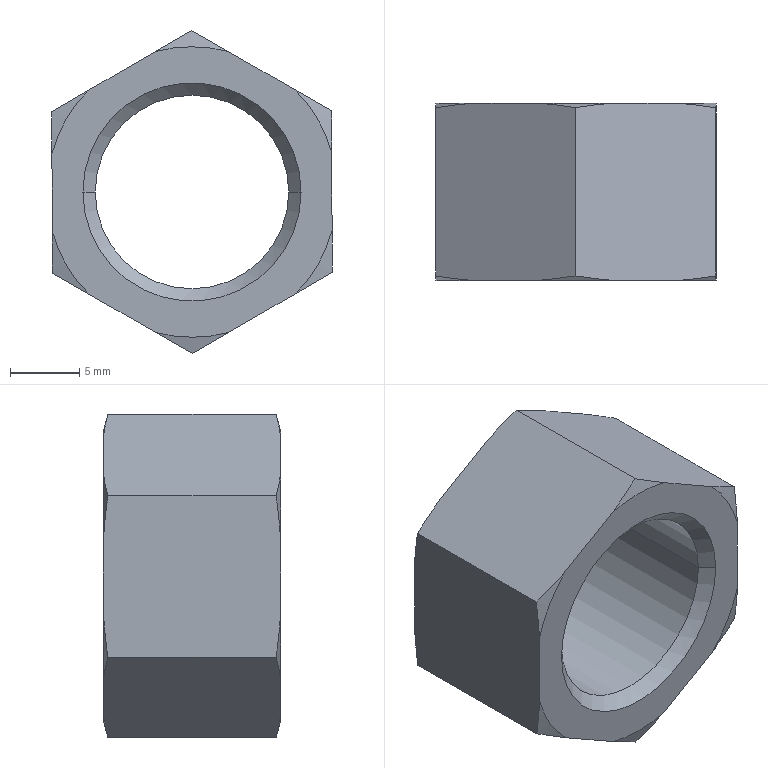Component | SolidWorks | 25Type1HexNut_GradeAAndB[GBT6170-2000][M14]-2 | 1 solid | 26 faces | box 20.28 x 12.8 x 23.36 mm | volume 2527 mm3 | cone 16 | plane 8 | cylinder 2 | commonest cylinder face diameters 14 x2 | material Steel
STEP:
#1=COLOUR_RGB('',0.7922,0.8196,0.9333);
#2=FILL_AREA_STYLE_COLOUR('',#1);
#3=FILL_AREA_STYLE('',(#2));
#4=SURFACE_STYLE_FILL_AREA(#3);
#5=SURFACE_SIDE_STYLE('',(#4));
#6=SURFACE_STYLE_USAGE(.BOTH.,#5);
#7=PRESENTATION_STYLE_ASSIGNMENT((#6));
#8=CARTESIAN_POINT('',(4.247,3.56,16.299));
#9=VERTEX_POINT('',#8);
#10=CARTESIAN_POINT('',(4.799,3.56,16.299));
#11=VERTEX_POINT('',#10);
#12=CARTESIAN_POINT('',(4.523,3.56,16.299));
#13=DIRECTION('',(-0.,1.,0.));
#14=DIRECTION('',(-1.,0.,0.));
#15=AXIS2_PLACEMENT_3D('',#12,#13,#14);
#16=CIRCLE('',#15,0.2756);
#17=EDGE_CURVE('',#9,#11,#16,.T.);
#18=ORIENTED_EDGE('',*,*,#17,.F.);
#19=CARTESIAN_POINT('',(4.213,3.595,16.299));
#20=VERTEX_POINT('',#19);
#21=CARTESIAN_POINT('',(4.247,3.56,16.299));
#22=DIRECTION('',(-0.7071,0.7071,-0.));
#23=VECTOR('',#22,39.37);
#24=LINE('',#21,#23);
#25=EDGE_CURVE('',#9,#20,#24,.T.);
#26=ORIENTED_EDGE('',*,*,#25,.T.);
#27=CARTESIAN_POINT('',(4.833,3.595,16.299));
#28=VERTEX_POINT('',#27);
#29=CARTESIAN_POINT('',(4.523,3.595,16.299));
#30=DIRECTION('',(0.,-1.,0.));
#31=DIRECTION('',(-1.,0.,0.));
#32=AXIS2_PLACEMENT_3D('',#29,#30,#31);
#33=CIRCLE('',#32,0.3104);
#34=EDGE_CURVE('',#28,#20,#33,.T.);
#35=ORIENTED_EDGE('',*,*,#34,.F.);
#36=CARTESIAN_POINT('',(4.799,3.56,16.299));
#37=DIRECTION('',(0.7071,0.7071,0.));
#38=VECTOR('',#37,39.37);
#39=LINE('',#36,#38);
#40=EDGE_CURVE('',#11,#28,#39,.T.);
#41=ORIENTED_EDGE('',*,*,#40,.F.);
#42=EDGE_LOOP('',(#18,#26,#35,#41));
#43=FACE_OUTER_BOUND('',#42,.T.);
#44=CARTESIAN_POINT('',(4.523,3.56,16.299));
#45=DIRECTION('',(-0.,1.,0.));
#46=DIRECTION('',(1.,0.,0.));
#47=AXIS2_PLACEMENT_3D('',#44,#45,#46);
#48=CONICAL_SURFACE('',#47,0.2756,0.7854);
#49=ADVANCED_FACE('',(#43),#48,.F.);
#50=CARTESIAN_POINT('',(4.799,3.126,16.299));
#51=VERTEX_POINT('',#50);
#52=CARTESIAN_POINT('',(4.247,3.126,16.299));
#53=VERTEX_POINT('',#52);
#54=CARTESIAN_POINT('',(4.523,3.126,16.299));
#55=DIRECTION('',(0.,-1.,0.));
#56=DIRECTION('',(-1.,0.,0.));
#57=AXIS2_PLACEMENT_3D('',#54,#55,#56);
#58=CIRCLE('',#57,0.2756);
#59=EDGE_CURVE('',#51,#53,#58,.T.);
#60=ORIENTED_EDGE('',*,*,#59,.F.);
#61=CARTESIAN_POINT('',(4.833,3.091,16.299));
#62=VERTEX_POINT('',#61);
#63=CARTESIAN_POINT('',(4.833,3.091,16.299));
#64=DIRECTION('',(0.7071,-0.7071,-0.));
#65=VECTOR('',#64,39.37);
#66=LINE('',#63,#65);
#67=EDGE_CURVE('',#51,#62,#66,.T.);
#68=ORIENTED_EDGE('',*,*,#67,.T.);
#69=CARTESIAN_POINT('',(4.213,3.091,16.299));
#70=VERTEX_POINT('',#69);
#71=CARTESIAN_POINT('',(4.523,3.091,16.299));
#72=DIRECTION('',(-0.,1.,0.));
#73=DIRECTION('',(-1.,0.,0.));
#74=AXIS2_PLACEMENT_3D('',#71,#72,#73);
#75=CIRCLE('',#74,0.3104);
#76=EDGE_CURVE('',#70,#62,#75,.T.);
#77=ORIENTED_EDGE('',*,*,#76,.F.);
#78=CARTESIAN_POINT('',(4.213,3.091,16.299));
#79=DIRECTION('',(-0.7071,-0.7071,-0.));
#80=VECTOR('',#79,39.37);
#81=LINE('',#78,#80);
#82=EDGE_CURVE('',#53,#70,#81,.T.);
#83=ORIENTED_EDGE('',*,*,#82,.F.);
#84=EDGE_LOOP('',(#60,#68,#77,#83));
#85=FACE_OUTER_BOUND('',#84,.T.);
#86=CARTESIAN_POINT('',(4.523,3.091,16.299));
#87=DIRECTION('',(0.,-1.,0.));
#88=DIRECTION('',(-1.,0.,0.));
#89=AXIS2_PLACEMENT_3D('',#86,#87,#88);
#90=CONICAL_SURFACE('',#89,0.3104,0.7854);
#91=ADVANCED_FACE('',(#85),#90,.F.);
#92=ORIENTED_EDGE('',*,*,#17,.T.);
#93=CARTESIAN_POINT('',(4.799,3.595,16.299));
#94=DIRECTION('',(0.,-1.,0.));
#95=VECTOR('',#94,39.37);
#96=LINE('',#93,#95);
#97=EDGE_CURVE('',#11,#51,#96,.T.);
#98=ORIENTED_EDGE('',*,*,#97,.T.);
#99=ORIENTED_EDGE('',*,*,#59,.T.);
#100=CARTESIAN_POINT('',(4.247,3.595,16.299));
#101=DIRECTION('',(0.,-1.,0.));
#102=VECTOR('',#101,39.37);
#103=LINE('',#100,#102);
#104=EDGE_CURVE('',#9,#53,#103,.T.);
#105=ORIENTED_EDGE('',*,*,#104,.F.);
#106=EDGE_LOOP('',(#92,#98,#99,#105));
#107=FACE_OUTER_BOUND('',#106,.T.);
#108=CARTESIAN_POINT('',(4.523,3.595,16.299));
#109=DIRECTION('',(0.,-1.,0.));
#110=DIRECTION('',(-1.,0.,0.));
#111=AXIS2_PLACEMENT_3D('',#108,#109,#110);
#112=CYLINDRICAL_SURFACE('',#111,0.2756);
#113=ADVANCED_FACE('',(#107),#112,.F.);
#114=CARTESIAN_POINT('',(4.922,3.582,16.071));
#115=VERTEX_POINT('',#114);
#116=CARTESIAN_POINT('',(4.819,3.595,16.011));
#117=VERTEX_POINT('',#116);
#118=CARTESIAN_POINT('',(4.922,3.582,16.071));
#119=CARTESIAN_POINT('',(4.888,3.588,16.051));
#120=CARTESIAN_POINT('',(4.854,3.592,16.031));
#121=CARTESIAN_POINT('',(4.819,3.595,16.011));
#122=B_SPLINE_CURVE_WITH_KNOTS('',3,(#118,#119,#120,#121),.UNSPECIFIED.,.F.,.F.,(4,4),(0.01194,0.01498),.UNSPECIFIED.);
#123=EDGE_CURVE('',#115,#117,#122,.T.);
#124=ORIENTED_EDGE('',*,*,#123,.F.);
#125=CARTESIAN_POINT('',(4.922,3.103,16.071));
#126=VERTEX_POINT('',#125);
#127=CARTESIAN_POINT('',(4.922,3.595,16.071));
#128=DIRECTION('',(0.,-1.,0.));
#129=VECTOR('',#128,39.37);
#130=LINE('',#127,#129);
#131=EDGE_CURVE('',#115,#126,#130,.T.);
#132=ORIENTED_EDGE('',*,*,#131,.T.);
#133=CARTESIAN_POINT('',(4.819,3.091,16.011));
#134=VERTEX_POINT('',#133);
#135=CARTESIAN_POINT('',(4.819,3.091,16.011));
#136=CARTESIAN_POINT('',(4.854,3.094,16.031));
#137=CARTESIAN_POINT('',(4.888,3.098,16.051));
#138=CARTESIAN_POINT('',(4.922,3.103,16.071));
#139=B_SPLINE_CURVE_WITH_KNOTS('',3,(#135,#136,#137,#138),.UNSPECIFIED.,.F.,.F.,(4,4),(0.02057,0.02356),.UNSPECIFIED.);
#140=EDGE_CURVE('',#134,#126,#139,.T.);
#141=ORIENTED_EDGE('',*,*,#140,.F.);
#142=CARTESIAN_POINT('',(4.628,3.091,15.899));
#143=VERTEX_POINT('',#142);
#144=CARTESIAN_POINT('',(4.922,3.091,16.071));
#145=DIRECTION('',(-0.8641,-0.,-0.5034));
#146=VECTOR('',#145,39.37);
#147=LINE('',#144,#146);
#148=EDGE_CURVE('',#134,#143,#147,.T.);
#149=ORIENTED_EDGE('',*,*,#148,.T.);
#150=CARTESIAN_POINT('',(4.525,3.103,15.839));
#151=VERTEX_POINT('',#150);
#152=CARTESIAN_POINT('',(4.525,3.103,15.839));
#153=CARTESIAN_POINT('',(4.559,3.098,15.859));
#154=CARTESIAN_POINT('',(4.593,3.094,15.879));
#155=CARTESIAN_POINT('',(4.628,3.091,15.899));
#156=B_SPLINE_CURVE_WITH_KNOTS('',3,(#152,#153,#154,#155),.UNSPECIFIED.,.F.,.F.,(4,4),(0.01194,0.01498),.UNSPECIFIED.);
#157=EDGE_CURVE('',#151,#143,#156,.T.);
#158=ORIENTED_EDGE('',*,*,#157,.F.);
#159=CARTESIAN_POINT('',(4.525,3.582,15.839));
#160=VERTEX_POINT('',#159);
#161=CARTESIAN_POINT('',(4.525,3.595,15.839));
#162=DIRECTION('',(0.,-1.,0.));
#163=VECTOR('',#162,39.37);
#164=LINE('',#161,#163);
#165=EDGE_CURVE('',#160,#151,#164,.T.);
#166=ORIENTED_EDGE('',*,*,#165,.F.);
#167=CARTESIAN_POINT('',(4.628,3.595,15.899));
#168=VERTEX_POINT('',#167);
#169=CARTESIAN_POINT('',(4.628,3.595,15.899));
#170=CARTESIAN_POINT('',(4.593,3.592,15.879));
#171=CARTESIAN_POINT('',(4.559,3.588,15.859));
#172=CARTESIAN_POINT('',(4.525,3.582,15.839));
#173=B_SPLINE_CURVE_WITH_KNOTS('',3,(#169,#170,#171,#172),.UNSPECIFIED.,.F.,.F.,(4,4),(0.02057,0.02356),.UNSPECIFIED.);
#174=EDGE_CURVE('',#168,#160,#173,.T.);
#175=ORIENTED_EDGE('',*,*,#174,.F.);
#176=CARTESIAN_POINT('',(4.922,3.595,16.071));
#177=DIRECTION('',(-0.8641,-0.,-0.5034));
#178=VECTOR('',#177,39.37);
#179=LINE('',#176,#178);
#180=EDGE_CURVE('',#117,#168,#179,.T.);
#181=ORIENTED_EDGE('',*,*,#180,.F.);
#182=EDGE_LOOP('',(#124,#132,#141,#149,#158,#166,#175,#181));
#183=FACE_OUTER_BOUND('',#182,.T.);
#184=CARTESIAN_POINT('',(4.922,3.595,16.071));
#185=DIRECTION('',(-0.5034,-0.,0.8641));
#186=DIRECTION('',(0.8641,0.,0.5034));
#187=AXIS2_PLACEMENT_3D('',#184,#185,#186);
#188=PLANE('',#187);
#189=ADVANCED_FACE('',(#183),#188,.F.);
#190=CARTESIAN_POINT('',(4.422,3.595,15.898));
#191=VERTEX_POINT('',#190);
#192=CARTESIAN_POINT('',(4.525,3.582,15.839));
#193=CARTESIAN_POINT('',(4.491,3.588,15.859));
#194=CARTESIAN_POINT('',(4.456,3.592,15.879));
#195=CARTESIAN_POINT('',(4.422,3.595,15.898));
#196=B_SPLINE_CURVE_WITH_KNOTS('',3,(#192,#193,#194,#195),.UNSPECIFIED.,.F.,.F.,(4,4),(0.01189,0.01493),.UNSPECIFIED.);
#197=EDGE_CURVE('',#160,#191,#196,.T.);
#198=ORIENTED_EDGE('',*,*,#197,.F.);
#199=ORIENTED_EDGE('',*,*,#165,.T.);
#200=CARTESIAN_POINT('',(4.422,3.091,15.898));
#201=VERTEX_POINT('',#200);
#202=CARTESIAN_POINT('',(4.422,3.091,15.898));
#203=CARTESIAN_POINT('',(4.456,3.094,15.879));
#204=CARTESIAN_POINT('',(4.491,3.098,15.859));
#205=CARTESIAN_POINT('',(4.525,3.103,15.839));
#206=B_SPLINE_CURVE_WITH_KNOTS('',3,(#202,#203,#204,#205),.UNSPECIFIED.,.F.,.F.,(4,4),(0.02052,0.0235),.UNSPECIFIED.);
#207=EDGE_CURVE('',#201,#151,#206,.T.);
#208=ORIENTED_EDGE('',*,*,#207,.F.);
#209=CARTESIAN_POINT('',(4.229,3.091,16.009));
#210=VERTEX_POINT('',#209);
#211=CARTESIAN_POINT('',(4.525,3.091,15.839));
#212=DIRECTION('',(-0.868,-0.,0.4966));
#213=VECTOR('',#212,39.37);
#214=LINE('',#211,#213);
#215=EDGE_CURVE('',#201,#210,#214,.T.);
#216=ORIENTED_EDGE('',*,*,#215,.T.);
#217=CARTESIAN_POINT('',(4.126,3.103,16.068));
#218=VERTEX_POINT('',#217);
#219=CARTESIAN_POINT('',(4.126,3.103,16.068));
#220=CARTESIAN_POINT('',(4.16,3.098,16.048));
#221=CARTESIAN_POINT('',(4.194,3.094,16.028));
#222=CARTESIAN_POINT('',(4.229,3.091,16.009));
#223=B_SPLINE_CURVE_WITH_KNOTS('',3,(#219,#220,#221,#222),.UNSPECIFIED.,.F.,.F.,(4,4),(0.01189,0.01493),.UNSPECIFIED.);
#224=EDGE_CURVE('',#218,#210,#223,.T.);
#225=ORIENTED_EDGE('',*,*,#224,.F.);
#226=CARTESIAN_POINT('',(4.126,3.582,16.068));
#227=VERTEX_POINT('',#226);
#228=CARTESIAN_POINT('',(4.126,3.595,16.068));
#229=DIRECTION('',(0.,-1.,0.));
#230=VECTOR('',#229,39.37);
#231=LINE('',#228,#230);
#232=EDGE_CURVE('',#227,#218,#231,.T.);
#233=ORIENTED_EDGE('',*,*,#232,.F.);
#234=CARTESIAN_POINT('',(4.229,3.595,16.009));
#235=VERTEX_POINT('',#234);
#236=CARTESIAN_POINT('',(4.229,3.595,16.009));
#237=CARTESIAN_POINT('',(4.194,3.592,16.028));
#238=CARTESIAN_POINT('',(4.16,3.588,16.048));
#239=CARTESIAN_POINT('',(4.126,3.582,16.068));
#240=B_SPLINE_CURVE_WITH_KNOTS('',3,(#236,#237,#238,#239),.UNSPECIFIED.,.F.,.F.,(4,4),(0.02052,0.0235),.UNSPECIFIED.);
#241=EDGE_CURVE('',#235,#227,#240,.T.);
#242=ORIENTED_EDGE('',*,*,#241,.F.);
#243=CARTESIAN_POINT('',(4.525,3.595,15.839));
#244=DIRECTION('',(-0.868,-0.,0.4966));
#245=VECTOR('',#244,39.37);
#246=LINE('',#243,#245);
#247=EDGE_CURVE('',#191,#235,#246,.T.);
#248=ORIENTED_EDGE('',*,*,#247,.F.);
#249=EDGE_LOOP('',(#198,#199,#208,#216,#225,#233,#242,#248));
#250=FACE_OUTER_BOUND('',#249,.T.);
#251=CARTESIAN_POINT('',(4.525,3.595,15.839));
#252=DIRECTION('',(0.4966,0.,0.868));
#253=DIRECTION('',(0.868,0.,-0.4966));
#254=AXIS2_PLACEMENT_3D('',#251,#252,#253);
#255=PLANE('',#254);
#256=ADVANCED_FACE('',(#250),#255,.F.);
#257=CARTESIAN_POINT('',(4.125,3.595,16.187));
#258=VERTEX_POINT('',#257);
#259=CARTESIAN_POINT('',(4.126,3.582,16.068));
#260=CARTESIAN_POINT('',(4.126,3.588,16.107));
#261=CARTESIAN_POINT('',(4.125,3.592,16.147));
#262=CARTESIAN_POINT('',(4.125,3.595,16.187));
#263=B_SPLINE_CURVE_WITH_KNOTS('',3,(#259,#260,#261,#262),.UNSPECIFIED.,.F.,.F.,(4,4),(0.01031,0.01335),.UNSPECIFIED.);
#264=EDGE_CURVE('',#227,#258,#263,.T.);
#265=ORIENTED_EDGE('',*,*,#264,.F.);
#266=ORIENTED_EDGE('',*,*,#232,.T.);
#267=CARTESIAN_POINT('',(4.125,3.091,16.187));
#268=VERTEX_POINT('',#267);
#269=CARTESIAN_POINT('',(4.125,3.091,16.187));
#270=CARTESIAN_POINT('',(4.125,3.094,16.147));
#271=CARTESIAN_POINT('',(4.126,3.098,16.107));
#272=CARTESIAN_POINT('',(4.126,3.103,16.068));
#273=B_SPLINE_CURVE_WITH_KNOTS('',3,(#269,#270,#271,#272),.UNSPECIFIED.,.F.,.F.,(4,4),(0.01894,0.02193),.UNSPECIFIED.);
#274=EDGE_CURVE('',#268,#218,#273,.T.);
#275=ORIENTED_EDGE('',*,*,#274,.F.);
#276=CARTESIAN_POINT('',(4.124,3.091,16.409));
#277=VERTEX_POINT('',#276);
#278=CARTESIAN_POINT('',(4.126,3.091,16.068));
#279=DIRECTION('',(-0.003934,-0.,1.));
#280=VECTOR('',#279,39.37);
#281=LINE('',#278,#280);
#282=EDGE_CURVE('',#268,#277,#281,.T.);
#283=ORIENTED_EDGE('',*,*,#282,.T.);
#284=CARTESIAN_POINT('',(4.124,3.103,16.528));
#285=VERTEX_POINT('',#284);
#286=CARTESIAN_POINT('',(4.124,3.103,16.528));
#287=CARTESIAN_POINT('',(4.124,3.098,16.488));
#288=CARTESIAN_POINT('',(4.124,3.094,16.448));
#289=CARTESIAN_POINT('',(4.124,3.091,16.409));
#290=B_SPLINE_CURVE_WITH_KNOTS('',3,(#286,#287,#288,#289),.UNSPECIFIED.,.F.,.F.,(4,4),(0.01031,0.01335),.UNSPECIFIED.);
#291=EDGE_CURVE('',#285,#277,#290,.T.);
#292=ORIENTED_EDGE('',*,*,#291,.F.);
#293=CARTESIAN_POINT('',(4.124,3.582,16.528));
#294=VERTEX_POINT('',#293);
#295=CARTESIAN_POINT('',(4.124,3.595,16.528));
#296=DIRECTION('',(0.,-1.,0.));
#297=VECTOR('',#296,39.37);
#298=LINE('',#295,#297);
#299=EDGE_CURVE('',#294,#285,#298,.T.);
#300=ORIENTED_EDGE('',*,*,#299,.F.);
#301=CARTESIAN_POINT('',(4.124,3.595,16.409));
#302=VERTEX_POINT('',#301);
#303=CARTESIAN_POINT('',(4.124,3.595,16.409));
#304=CARTESIAN_POINT('',(4.124,3.592,16.448));
#305=CARTESIAN_POINT('',(4.124,3.588,16.488));
#306=CARTESIAN_POINT('',(4.124,3.582,16.528));
#307=B_SPLINE_CURVE_WITH_KNOTS('',3,(#303,#304,#305,#306),.UNSPECIFIED.,.F.,.F.,(4,4),(0.01894,0.02193),.UNSPECIFIED.);
#308=EDGE_CURVE('',#302,#294,#307,.T.);
#309=ORIENTED_EDGE('',*,*,#308,.F.);
#310=CARTESIAN_POINT('',(4.126,3.595,16.068));
#311=DIRECTION('',(-0.003934,-0.,1.));
#312=VECTOR('',#311,39.37);
#313=LINE('',#310,#312);
#314=EDGE_CURVE('',#258,#302,#313,.T.);
#315=ORIENTED_EDGE('',*,*,#314,.F.);
#316=EDGE_LOOP('',(#265,#266,#275,#283,#292,#300,#309,#315));
#317=FACE_OUTER_BOUND('',#316,.T.);
#318=CARTESIAN_POINT('',(4.126,3.595,16.068));
#319=DIRECTION('',(1.,0.,0.003934));
#320=DIRECTION('',(0.003934,0.,-1.));
#321=AXIS2_PLACEMENT_3D('',#318,#319,#320);
#322=PLANE('',#321);
#323=ADVANCED_FACE('',(#317),#322,.F.);
#324=CARTESIAN_POINT('',(4.227,3.595,16.587));
#325=VERTEX_POINT('',#324);
#326=CARTESIAN_POINT('',(4.124,3.582,16.528));
#327=CARTESIAN_POINT('',(4.158,3.588,16.547));
#328=CARTESIAN_POINT('',(4.192,3.592,16.567));
#329=CARTESIAN_POINT('',(4.227,3.595,16.587));
#330=B_SPLINE_CURVE_WITH_KNOTS('',3,(#326,#327,#328,#329),.UNSPECIFIED.,.F.,.F.,(4,4),(0.01194,0.01498),.UNSPECIFIED.);
#331=EDGE_CURVE('',#294,#325,#330,.T.);
#332=ORIENTED_EDGE('',*,*,#331,.F.);
#333=ORIENTED_EDGE('',*,*,#299,.T.);
#334=CARTESIAN_POINT('',(4.227,3.091,16.587));
#335=VERTEX_POINT('',#334);
#336=CARTESIAN_POINT('',(4.227,3.091,16.587));
#337=CARTESIAN_POINT('',(4.192,3.094,16.567));
#338=CARTESIAN_POINT('',(4.158,3.098,16.547));
#339=CARTESIAN_POINT('',(4.124,3.103,16.528));
#340=B_SPLINE_CURVE_WITH_KNOTS('',3,(#336,#337,#338,#339),.UNSPECIFIED.,.F.,.F.,(4,4),(0.02057,0.02356),.UNSPECIFIED.);
#341=EDGE_CURVE('',#335,#285,#340,.T.);
#342=ORIENTED_EDGE('',*,*,#341,.F.);
#343=CARTESIAN_POINT('',(4.418,3.091,16.699));
#344=VERTEX_POINT('',#343);
#345=CARTESIAN_POINT('',(4.124,3.091,16.528));
#346=DIRECTION('',(0.8641,0.,0.5034));
#347=VECTOR('',#346,39.37);
#348=LINE('',#345,#347);
#349=EDGE_CURVE('',#335,#344,#348,.T.);
#350=ORIENTED_EDGE('',*,*,#349,.T.);
#351=CARTESIAN_POINT('',(4.521,3.103,16.759));
#352=VERTEX_POINT('',#351);
#353=CARTESIAN_POINT('',(4.521,3.103,16.759));
#354=CARTESIAN_POINT('',(4.487,3.098,16.739));
#355=CARTESIAN_POINT('',(4.453,3.094,16.719));
#356=CARTESIAN_POINT('',(4.418,3.091,16.699));
#357=B_SPLINE_CURVE_WITH_KNOTS('',3,(#353,#354,#355,#356),.UNSPECIFIED.,.F.,.F.,(4,4),(0.01194,0.01498),.UNSPECIFIED.);
#358=EDGE_CURVE('',#352,#344,#357,.T.);
#359=ORIENTED_EDGE('',*,*,#358,.F.);
#360=CARTESIAN_POINT('',(4.521,3.582,16.759));
#361=VERTEX_POINT('',#360);
#362=CARTESIAN_POINT('',(4.521,3.595,16.759));
#363=DIRECTION('',(0.,-1.,0.));
#364=VECTOR('',#363,39.37);
#365=LINE('',#362,#364);
#366=EDGE_CURVE('',#361,#352,#365,.T.);
#367=ORIENTED_EDGE('',*,*,#366,.F.);
#368=CARTESIAN_POINT('',(4.418,3.595,16.699));
#369=VERTEX_POINT('',#368);
#370=CARTESIAN_POINT('',(4.418,3.595,16.699));
#371=CARTESIAN_POINT('',(4.453,3.592,16.719));
#372=CARTESIAN_POINT('',(4.487,3.588,16.739));
#373=CARTESIAN_POINT('',(4.521,3.582,16.759));
#374=B_SPLINE_CURVE_WITH_KNOTS('',3,(#370,#371,#372,#373),.UNSPECIFIED.,.F.,.F.,(4,4),(0.02057,0.02356),.UNSPECIFIED.);
#375=EDGE_CURVE('',#369,#361,#374,.T.);
#376=ORIENTED_EDGE('',*,*,#375,.F.);
#377=CARTESIAN_POINT('',(4.124,3.595,16.528));
#378=DIRECTION('',(0.8641,0.,0.5034));
#379=VECTOR('',#378,39.37);
#380=LINE('',#377,#379);
#381=EDGE_CURVE('',#325,#369,#380,.T.);
#382=ORIENTED_EDGE('',*,*,#381,.F.);
#383=EDGE_LOOP('',(#332,#333,#342,#350,#359,#367,#376,#382));
#384=FACE_OUTER_BOUND('',#383,.T.);
#385=CARTESIAN_POINT('',(4.124,3.595,16.528));
#386=DIRECTION('',(0.5034,0.,-0.8641));
#387=DIRECTION('',(-0.8641,-0.,-0.5034));
#388=AXIS2_PLACEMENT_3D('',#385,#386,#387);
#389=PLANE('',#388);
#390=ADVANCED_FACE('',(#384),#389,.F.);
#391=CARTESIAN_POINT('',(4.625,3.595,16.7));
#392=VERTEX_POINT('',#391);
#393=CARTESIAN_POINT('',(4.521,3.582,16.759));
#394=CARTESIAN_POINT('',(4.556,3.588,16.739));
#395=CARTESIAN_POINT('',(4.59,3.592,16.72));
#396=CARTESIAN_POINT('',(4.625,3.595,16.7));
#397=B_SPLINE_CURVE_WITH_KNOTS('',3,(#393,#394,#395,#396),.UNSPECIFIED.,.F.,.F.,(4,4),(0.01189,0.01493),.UNSPECIFIED.);
#398=EDGE_CURVE('',#361,#392,#397,.T.);
#399=ORIENTED_EDGE('',*,*,#398,.F.);
#400=ORIENTED_EDGE('',*,*,#366,.T.);
#401=CARTESIAN_POINT('',(4.625,3.091,16.7));
#402=VERTEX_POINT('',#401);
#403=CARTESIAN_POINT('',(4.625,3.091,16.7));
#404=CARTESIAN_POINT('',(4.59,3.094,16.72));
#405=CARTESIAN_POINT('',(4.555,3.098,16.739));
#406=CARTESIAN_POINT('',(4.521,3.103,16.759));
#407=B_SPLINE_CURVE_WITH_KNOTS('',3,(#403,#404,#405,#406),.UNSPECIFIED.,.F.,.F.,(4,4),(0.02052,0.0235),.UNSPECIFIED.);
#408=EDGE_CURVE('',#402,#352,#407,.T.);
#409=ORIENTED_EDGE('',*,*,#408,.F.);
#410=CARTESIAN_POINT('',(4.817,3.091,16.59));
#411=VERTEX_POINT('',#410);
#412=CARTESIAN_POINT('',(4.521,3.091,16.759));
#413=DIRECTION('',(0.868,0.,-0.4966));
#414=VECTOR('',#413,39.37);
#415=LINE('',#412,#414);
#416=EDGE_CURVE('',#402,#411,#415,.T.);
#417=ORIENTED_EDGE('',*,*,#416,.T.);
#418=CARTESIAN_POINT('',(4.92,3.103,16.531));
#419=VERTEX_POINT('',#418);
#420=CARTESIAN_POINT('',(4.92,3.103,16.531));
#421=CARTESIAN_POINT('',(4.886,3.098,16.55));
#422=CARTESIAN_POINT('',(4.852,3.094,16.57));
#423=CARTESIAN_POINT('',(4.817,3.091,16.59));
#424=B_SPLINE_CURVE_WITH_KNOTS('',3,(#420,#421,#422,#423),.UNSPECIFIED.,.F.,.F.,(4,4),(0.01189,0.01493),.UNSPECIFIED.);
#425=EDGE_CURVE('',#419,#411,#424,.T.);
#426=ORIENTED_EDGE('',*,*,#425,.F.);
#427=CARTESIAN_POINT('',(4.92,3.582,16.531));
#428=VERTEX_POINT('',#427);
#429=CARTESIAN_POINT('',(4.92,3.595,16.531));
#430=DIRECTION('',(0.,-1.,0.));
#431=VECTOR('',#430,39.37);
#432=LINE('',#429,#431);
#433=EDGE_CURVE('',#428,#419,#432,.T.);
#434=ORIENTED_EDGE('',*,*,#433,.F.);
#435=CARTESIAN_POINT('',(4.817,3.595,16.59));
#436=VERTEX_POINT('',#435);
#437=CARTESIAN_POINT('',(4.817,3.595,16.59));
#438=CARTESIAN_POINT('',(4.852,3.592,16.57));
#439=CARTESIAN_POINT('',(4.886,3.588,16.55));
#440=CARTESIAN_POINT('',(4.92,3.582,16.531));
#441=B_SPLINE_CURVE_WITH_KNOTS('',3,(#437,#438,#439,#440),.UNSPECIFIED.,.F.,.F.,(4,4),(0.02052,0.0235),.UNSPECIFIED.);
#442=EDGE_CURVE('',#436,#428,#441,.T.);
#443=ORIENTED_EDGE('',*,*,#442,.F.);
#444=CARTESIAN_POINT('',(4.521,3.595,16.759));
#445=DIRECTION('',(0.868,0.,-0.4966));
#446=VECTOR('',#445,39.37);
#447=LINE('',#444,#446);
#448=EDGE_CURVE('',#392,#436,#447,.T.);
#449=ORIENTED_EDGE('',*,*,#448,.F.);
#450=EDGE_LOOP('',(#399,#400,#409,#417,#426,#434,#443,#449));
#451=FACE_OUTER_BOUND('',#450,.T.);
#452=CARTESIAN_POINT('',(4.521,3.595,16.759));
#453=DIRECTION('',(-0.4966,-0.,-0.868));
#454=DIRECTION('',(-0.868,-0.,0.4966));
#455=AXIS2_PLACEMENT_3D('',#452,#453,#454);
#456=PLANE('',#455);
#457=ADVANCED_FACE('',(#451),#456,.F.);
#458=CARTESIAN_POINT('',(4.921,3.595,16.412));
#459=VERTEX_POINT('',#458);
#460=CARTESIAN_POINT('',(4.92,3.582,16.531));
#461=CARTESIAN_POINT('',(4.921,3.588,16.491));
#462=CARTESIAN_POINT('',(4.921,3.592,16.451));
#463=CARTESIAN_POINT('',(4.921,3.595,16.412));
#464=B_SPLINE_CURVE_WITH_KNOTS('',3,(#460,#461,#462,#463),.UNSPECIFIED.,.F.,.F.,(4,4),(0.01031,0.01335),.UNSPECIFIED.);
#465=EDGE_CURVE('',#428,#459,#464,.T.);
#466=ORIENTED_EDGE('',*,*,#465,.F.);
#467=ORIENTED_EDGE('',*,*,#433,.T.);
#468=CARTESIAN_POINT('',(4.921,3.091,16.412));
#469=VERTEX_POINT('',#468);
#470=CARTESIAN_POINT('',(4.921,3.091,16.412));
#471=CARTESIAN_POINT('',(4.921,3.094,16.451));
#472=CARTESIAN_POINT('',(4.921,3.098,16.491));
#473=CARTESIAN_POINT('',(4.92,3.103,16.531));
#474=B_SPLINE_CURVE_WITH_KNOTS('',3,(#470,#471,#472,#473),.UNSPECIFIED.,.F.,.F.,(4,4),(0.01894,0.02193),.UNSPECIFIED.);
#475=EDGE_CURVE('',#469,#419,#474,.T.);
#476=ORIENTED_EDGE('',*,*,#475,.F.);
#477=CARTESIAN_POINT('',(4.922,3.091,16.19));
#478=VERTEX_POINT('',#477);
#479=CARTESIAN_POINT('',(4.92,3.091,16.531));
#480=DIRECTION('',(0.003934,0.,-1.));
#481=VECTOR('',#480,39.37);
#482=LINE('',#479,#481);
#483=EDGE_CURVE('',#469,#478,#482,.T.);
#484=ORIENTED_EDGE('',*,*,#483,.T.);
#485=CARTESIAN_POINT('',(4.922,3.103,16.071));
#486=CARTESIAN_POINT('',(4.922,3.098,16.11));
#487=CARTESIAN_POINT('',(4.922,3.094,16.15));
#488=CARTESIAN_POINT('',(4.922,3.091,16.19));
#489=B_SPLINE_CURVE_WITH_KNOTS('',3,(#485,#486,#487,#488),.UNSPECIFIED.,.F.,.F.,(4,4),(0.01031,0.01335),.UNSPECIFIED.);
#490=EDGE_CURVE('',#126,#478,#489,.T.);
#491=ORIENTED_EDGE('',*,*,#490,.F.);
#492=ORIENTED_EDGE('',*,*,#131,.F.);
#493=CARTESIAN_POINT('',(4.922,3.595,16.19));
#494=VERTEX_POINT('',#493);
#495=CARTESIAN_POINT('',(4.922,3.595,16.19));
#496=CARTESIAN_POINT('',(4.922,3.592,16.15));
#497=CARTESIAN_POINT('',(4.922,3.588,16.11));
#498=CARTESIAN_POINT('',(4.922,3.582,16.071));
#499=B_SPLINE_CURVE_WITH_KNOTS('',3,(#495,#496,#497,#498),.UNSPECIFIED.,.F.,.F.,(4,4),(0.01894,0.02193),.UNSPECIFIED.);
#500=EDGE_CURVE('',#494,#115,#499,.T.);
#501=ORIENTED_EDGE('',*,*,#500,.F.);
#502=CARTESIAN_POINT('',(4.92,3.595,16.531));
#503=DIRECTION('',(0.003934,0.,-1.));
#504=VECTOR('',#503,39.37);
#505=LINE('',#502,#504);
#506=EDGE_CURVE('',#459,#494,#505,.T.);
#507=ORIENTED_EDGE('',*,*,#506,.F.);
#508=EDGE_LOOP('',(#466,#467,#476,#484,#491,#492,#501,#507));
#509=FACE_OUTER_BOUND('',#508,.T.);
#510=CARTESIAN_POINT('',(4.92,3.595,16.531));
#511=DIRECTION('',(-1.,-0.,-0.003934));
#512=DIRECTION('',(-0.003934,-0.,1.));
#513=AXIS2_PLACEMENT_3D('',#510,#511,#512);
#514=PLANE('',#513);
#515=ADVANCED_FACE('',(#509),#514,.F.);
#516=ORIENTED_EDGE('',*,*,#34,.T.);
#517=CARTESIAN_POINT('',(4.523,3.595,16.299));
#518=DIRECTION('',(0.,-1.,0.));
#519=DIRECTION('',(-1.,0.,0.));
#520=AXIS2_PLACEMENT_3D('',#517,#518,#519);
#521=CIRCLE('',#520,0.3104);
#522=EDGE_CURVE('',#20,#28,#521,.T.);
#523=ORIENTED_EDGE('',*,*,#522,.T.);
#524=EDGE_LOOP('',(#516,#523));
#525=FACE_BOUND('',#524,.T.);
#526=CARTESIAN_POINT('',(4.523,3.595,16.299));
#527=DIRECTION('',(0.,-1.,0.));
#528=DIRECTION('',(-1.,0.,0.));
#529=AXIS2_PLACEMENT_3D('',#526,#527,#528);
#530=CIRCLE('',#529,0.4134);
#531=EDGE_CURVE('',#258,#235,#530,.T.);
#532=ORIENTED_EDGE('',*,*,#531,.F.);
#533=ORIENTED_EDGE('',*,*,#314,.T.);
#534=CARTESIAN_POINT('',(4.523,3.595,16.299));
#535=DIRECTION('',(0.,-1.,0.));
#536=DIRECTION('',(-1.,0.,0.));
#537=AXIS2_PLACEMENT_3D('',#534,#535,#536);
#538=CIRCLE('',#537,0.4134);
#539=EDGE_CURVE('',#325,#302,#538,.T.);
#540=ORIENTED_EDGE('',*,*,#539,.F.);
#541=ORIENTED_EDGE('',*,*,#381,.T.);
#542=CARTESIAN_POINT('',(4.523,3.595,16.299));
#543=DIRECTION('',(0.,-1.,0.));
#544=DIRECTION('',(-1.,0.,0.));
#545=AXIS2_PLACEMENT_3D('',#542,#543,#544);
#546=CIRCLE('',#545,0.4134);
#547=EDGE_CURVE('',#392,#369,#546,.T.);
#548=ORIENTED_EDGE('',*,*,#547,.F.);
#549=ORIENTED_EDGE('',*,*,#448,.T.);
#550=CARTESIAN_POINT('',(4.523,3.595,16.299));
#551=DIRECTION('',(0.,-1.,0.));
#552=DIRECTION('',(-1.,0.,0.));
#553=AXIS2_PLACEMENT_3D('',#550,#551,#552);
#554=CIRCLE('',#553,0.4134);
#555=EDGE_CURVE('',#459,#436,#554,.T.);
#556=ORIENTED_EDGE('',*,*,#555,.F.);
#557=ORIENTED_EDGE('',*,*,#506,.T.);
#558=CARTESIAN_POINT('',(4.523,3.595,16.299));
#559=DIRECTION('',(-0.,1.,0.));
#560=DIRECTION('',(1.,0.,0.));
#561=AXIS2_PLACEMENT_3D('',#558,#559,#560);
#562=CIRCLE('',#561,0.4134);
#563=EDGE_CURVE('',#494,#117,#562,.T.);
#564=ORIENTED_EDGE('',*,*,#563,.T.);
#565=ORIENTED_EDGE('',*,*,#180,.T.);
#566=CARTESIAN_POINT('',(4.523,3.595,16.299));
#567=DIRECTION('',(0.,-1.,0.));
#568=DIRECTION('',(-1.,0.,0.));
#569=AXIS2_PLACEMENT_3D('',#566,#567,#568);
#570=CIRCLE('',#569,0.4134);
#571=EDGE_CURVE('',#191,#168,#570,.T.);
#572=ORIENTED_EDGE('',*,*,#571,.F.);
#573=ORIENTED_EDGE('',*,*,#247,.T.);
#574=EDGE_LOOP('',(#532,#533,#540,#541,#548,#549,#556,#557,#564,#565,#572,#573));
#575=FACE_OUTER_BOUND('',#574,.T.);
#576=CARTESIAN_POINT('',(4.922,3.595,16.071));
#577=DIRECTION('',(0.,-1.,0.));
#578=DIRECTION('',(-1.,-0.,-0.));
#579=AXIS2_PLACEMENT_3D('',#576,#577,#578);
#580=PLANE('',#579);
#581=ADVANCED_FACE('',(#525,#575),#580,.F.);
#582=ORIENTED_EDGE('',*,*,#76,.T.);
#583=CARTESIAN_POINT('',(4.523,3.091,16.299));
#584=DIRECTION('',(-0.,1.,0.));
#585=DIRECTION('',(-1.,0.,0.));
#586=AXIS2_PLACEMENT_3D('',#583,#584,#585);
#587=CIRCLE('',#586,0.3104);
#588=EDGE_CURVE('',#62,#70,#587,.T.);
#589=ORIENTED_EDGE('',*,*,#588,.T.);
#590=EDGE_LOOP('',(#582,#589));
#591=FACE_BOUND('',#590,.T.);
#592=ORIENTED_EDGE('',*,*,#282,.F.);
#593=CARTESIAN_POINT('',(4.523,3.091,16.299));
#594=DIRECTION('',(0.,-1.,0.));
#595=DIRECTION('',(-1.,0.,0.));
#596=AXIS2_PLACEMENT_3D('',#593,#594,#595);
#597=CIRCLE('',#596,0.4134);
#598=EDGE_CURVE('',#268,#210,#597,.T.);
#599=ORIENTED_EDGE('',*,*,#598,.T.);
#600=ORIENTED_EDGE('',*,*,#215,.F.);
#601=CARTESIAN_POINT('',(4.523,3.091,16.299));
#602=DIRECTION('',(0.,-1.,0.));
#603=DIRECTION('',(-1.,0.,0.));
#604=AXIS2_PLACEMENT_3D('',#601,#602,#603);
#605=CIRCLE('',#604,0.4134);
#606=EDGE_CURVE('',#201,#143,#605,.T.);
#607=ORIENTED_EDGE('',*,*,#606,.T.);
#608=ORIENTED_EDGE('',*,*,#148,.F.);
#609=CARTESIAN_POINT('',(4.523,3.091,16.299));
#610=DIRECTION('',(0.,-1.,0.));
#611=DIRECTION('',(-1.,0.,0.));
#612=AXIS2_PLACEMENT_3D('',#609,#610,#611);
#613=CIRCLE('',#612,0.4134);
#614=EDGE_CURVE('',#134,#478,#613,.T.);
#615=ORIENTED_EDGE('',*,*,#614,.T.);
#616=ORIENTED_EDGE('',*,*,#483,.F.);
#617=CARTESIAN_POINT('',(4.523,3.091,16.299));
#618=DIRECTION('',(0.,-1.,0.));
#619=DIRECTION('',(-1.,0.,0.));
#620=AXIS2_PLACEMENT_3D('',#617,#618,#619);
#621=CIRCLE('',#620,0.4134);
#622=EDGE_CURVE('',#469,#411,#621,.T.);
#623=ORIENTED_EDGE('',*,*,#622,.T.);
#624=ORIENTED_EDGE('',*,*,#416,.F.);
#625=CARTESIAN_POINT('',(4.523,3.091,16.299));
#626=DIRECTION('',(0.,-1.,0.));
#627=DIRECTION('',(-1.,0.,0.));
#628=AXIS2_PLACEMENT_3D('',#625,#626,#627);
#629=CIRCLE('',#628,0.4134);
#630=EDGE_CURVE('',#402,#344,#629,.T.);
#631=ORIENTED_EDGE('',*,*,#630,.T.);
#632=ORIENTED_EDGE('',*,*,#349,.F.);
#633=CARTESIAN_POINT('',(4.523,3.091,16.299));
#634=DIRECTION('',(0.,-1.,0.));
#635=DIRECTION('',(-1.,0.,0.));
#636=AXIS2_PLACEMENT_3D('',#633,#634,#635);
#637=CIRCLE('',#636,0.4134);
#638=EDGE_CURVE('',#335,#277,#637,.T.);
#639=ORIENTED_EDGE('',*,*,#638,.T.);
#640=EDGE_LOOP('',(#592,#599,#600,#607,#608,#615,#616,#623,#624,#631,#632,#639));
#641=FACE_OUTER_BOUND('',#640,.T.);
#642=CARTESIAN_POINT('',(4.922,3.091,16.071));
#643=DIRECTION('',(0.,-1.,0.));
#644=DIRECTION('',(-1.,-0.,-0.));
#645=AXIS2_PLACEMENT_3D('',#642,#643,#644);
#646=PLANE('',#645);
#647=ADVANCED_FACE('',(#591,#641),#646,.T.);
#648=ORIENTED_EDGE('',*,*,#97,.F.);
#649=CARTESIAN_POINT('',(4.523,3.56,16.299));
#650=DIRECTION('',(-0.,1.,0.));
#651=DIRECTION('',(-1.,0.,0.));
#652=AXIS2_PLACEMENT_3D('',#649,#650,#651);
#653=CIRCLE('',#652,0.2756);
#654=EDGE_CURVE('',#11,#9,#653,.T.);
#655=ORIENTED_EDGE('',*,*,#654,.T.);
#656=ORIENTED_EDGE('',*,*,#104,.T.);
#657=CARTESIAN_POINT('',(4.523,3.126,16.299));
#658=DIRECTION('',(0.,-1.,0.));
#659=DIRECTION('',(-1.,0.,0.));
#660=AXIS2_PLACEMENT_3D('',#657,#658,#659);
#661=CIRCLE('',#660,0.2756);
#662=EDGE_CURVE('',#53,#51,#661,.T.);
#663=ORIENTED_EDGE('',*,*,#662,.T.);
#664=EDGE_LOOP('',(#648,#655,#656,#663));
#665=FACE_OUTER_BOUND('',#664,.T.);
#666=CARTESIAN_POINT('',(4.523,3.595,16.299));
#667=DIRECTION('',(0.,-1.,0.));
#668=DIRECTION('',(-1.,0.,0.));
#669=AXIS2_PLACEMENT_3D('',#666,#667,#668);
#670=CYLINDRICAL_SURFACE('',#669,0.2756);
#671=ADVANCED_FACE('',(#665),#670,.F.);
#672=ORIENTED_EDGE('',*,*,#425,.T.);
#673=ORIENTED_EDGE('',*,*,#622,.F.);
#674=ORIENTED_EDGE('',*,*,#475,.T.);
#675=EDGE_LOOP('',(#672,#673,#674));
#676=FACE_OUTER_BOUND('',#675,.T.);
#677=CARTESIAN_POINT('',(4.523,3.091,16.299));
#678=DIRECTION('',(-0.,1.,0.));
#679=DIRECTION('',(-1.,0.,0.));
#680=AXIS2_PLACEMENT_3D('',#677,#678,#679);
#681=CONICAL_SURFACE('',#680,0.4134,1.309);
#682=ADVANCED_FACE('',(#676),#681,.T.);
#683=ORIENTED_EDGE('',*,*,#140,.T.);
#684=ORIENTED_EDGE('',*,*,#490,.T.);
#685=ORIENTED_EDGE('',*,*,#614,.F.);
#686=EDGE_LOOP('',(#683,#684,#685));
#687=FACE_OUTER_BOUND('',#686,.T.);
#688=CARTESIAN_POINT('',(4.523,3.091,16.299));
#689=DIRECTION('',(-0.,1.,0.));
#690=DIRECTION('',(-1.,0.,0.));
#691=AXIS2_PLACEMENT_3D('',#688,#689,#690);
#692=CONICAL_SURFACE('',#691,0.4134,1.309);
#693=ADVANCED_FACE('',(#687),#692,.T.);
#694=ORIENTED_EDGE('',*,*,#358,.T.);
#695=ORIENTED_EDGE('',*,*,#630,.F.);
#696=ORIENTED_EDGE('',*,*,#408,.T.);
#697=EDGE_LOOP('',(#694,#695,#696));
#698=FACE_OUTER_BOUND('',#697,.T.);
#699=CARTESIAN_POINT('',(4.523,3.091,16.299));
#700=DIRECTION('',(-0.,1.,0.));
#701=DIRECTION('',(-1.,0.,0.));
#702=AXIS2_PLACEMENT_3D('',#699,#700,#701);
#703=CONICAL_SURFACE('',#702,0.4134,1.309);
#704=ADVANCED_FACE('',(#698),#703,.T.);
#705=ORIENTED_EDGE('',*,*,#291,.T.);
#706=ORIENTED_EDGE('',*,*,#638,.F.);
#707=ORIENTED_EDGE('',*,*,#341,.T.);
#708=EDGE_LOOP('',(#705,#706,#707));
#709=FACE_OUTER_BOUND('',#708,.T.);
#710=CARTESIAN_POINT('',(4.523,3.091,16.299));
#711=DIRECTION('',(-0.,1.,0.));
#712=DIRECTION('',(-1.,0.,0.));
#713=AXIS2_PLACEMENT_3D('',#710,#711,#712);
#714=CONICAL_SURFACE('',#713,0.4134,1.309);
#715=ADVANCED_FACE('',(#709),#714,.T.);
#716=ORIENTED_EDGE('',*,*,#224,.T.);
#717=ORIENTED_EDGE('',*,*,#598,.F.);
#718=ORIENTED_EDGE('',*,*,#274,.T.);
#719=EDGE_LOOP('',(#716,#717,#718));
#720=FACE_OUTER_BOUND('',#719,.T.);
#721=CARTESIAN_POINT('',(4.523,3.091,16.299));
#722=DIRECTION('',(-0.,1.,0.));
#723=DIRECTION('',(-1.,0.,0.));
#724=AXIS2_PLACEMENT_3D('',#721,#722,#723);
#725=CONICAL_SURFACE('',#724,0.4134,1.309);
#726=ADVANCED_FACE('',(#720),#725,.T.);
#727=ORIENTED_EDGE('',*,*,#157,.T.);
#728=ORIENTED_EDGE('',*,*,#606,.F.);
#729=ORIENTED_EDGE('',*,*,#207,.T.);
#730=EDGE_LOOP('',(#727,#728,#729));
#731=FACE_OUTER_BOUND('',#730,.T.);
#732=CARTESIAN_POINT('',(4.523,3.091,16.299));
#733=DIRECTION('',(-0.,1.,0.));
#734=DIRECTION('',(-1.,0.,0.));
#735=AXIS2_PLACEMENT_3D('',#732,#733,#734);
#736=CONICAL_SURFACE('',#735,0.4134,1.309);
#737=ADVANCED_FACE('',(#731),#736,.T.);
#738=ORIENTED_EDGE('',*,*,#308,.T.);
#739=ORIENTED_EDGE('',*,*,#331,.T.);
#740=ORIENTED_EDGE('',*,*,#539,.T.);
#741=EDGE_LOOP('',(#738,#739,#740));
#742=FACE_OUTER_BOUND('',#741,.T.);
#743=CARTESIAN_POINT('',(4.523,3.595,16.299));
#744=DIRECTION('',(0.,-1.,0.));
#745=DIRECTION('',(1.,0.,0.));
#746=AXIS2_PLACEMENT_3D('',#743,#744,#745);
#747=CONICAL_SURFACE('',#746,0.4134,1.309);
#748=ADVANCED_FACE('',(#742),#747,.T.);
#749=ORIENTED_EDGE('',*,*,#375,.T.);
#750=ORIENTED_EDGE('',*,*,#398,.T.);
#751=ORIENTED_EDGE('',*,*,#547,.T.);
#752=EDGE_LOOP('',(#749,#750,#751));
#753=FACE_OUTER_BOUND('',#752,.T.);
#754=CARTESIAN_POINT('',(4.523,3.595,16.299));
#755=DIRECTION('',(0.,-1.,0.));
#756=DIRECTION('',(1.,0.,0.));
#757=AXIS2_PLACEMENT_3D('',#754,#755,#756);
#758=CONICAL_SURFACE('',#757,0.4134,1.309);
#759=ADVANCED_FACE('',(#753),#758,.T.);
#760=ORIENTED_EDGE('',*,*,#442,.T.);
#761=ORIENTED_EDGE('',*,*,#465,.T.);
#762=ORIENTED_EDGE('',*,*,#555,.T.);
#763=EDGE_LOOP('',(#760,#761,#762));
#764=FACE_OUTER_BOUND('',#763,.T.);
#765=CARTESIAN_POINT('',(4.523,3.595,16.299));
#766=DIRECTION('',(0.,-1.,0.));
#767=DIRECTION('',(1.,0.,0.));
#768=AXIS2_PLACEMENT_3D('',#765,#766,#767);
#769=CONICAL_SURFACE('',#768,0.4134,1.309);
#770=ADVANCED_FACE('',(#764),#769,.T.);
#771=ORIENTED_EDGE('',*,*,#123,.T.);
#772=ORIENTED_EDGE('',*,*,#563,.F.);
#773=ORIENTED_EDGE('',*,*,#500,.T.);
#774=EDGE_LOOP('',(#771,#772,#773));
#775=FACE_OUTER_BOUND('',#774,.T.);
#776=CARTESIAN_POINT('',(4.523,3.595,16.299));
#777=DIRECTION('',(0.,-1.,0.));
#778=DIRECTION('',(1.,0.,0.));
#779=AXIS2_PLACEMENT_3D('',#776,#777,#778);
#780=CONICAL_SURFACE('',#779,0.4134,1.309);
#781=ADVANCED_FACE('',(#775),#780,.T.);
#782=ORIENTED_EDGE('',*,*,#174,.T.);
#783=ORIENTED_EDGE('',*,*,#197,.T.);
#784=ORIENTED_EDGE('',*,*,#571,.T.);
#785=EDGE_LOOP('',(#782,#783,#784));
#786=FACE_OUTER_BOUND('',#785,.T.);
#787=CARTESIAN_POINT('',(4.523,3.595,16.299));
#788=DIRECTION('',(0.,-1.,0.));
#789=DIRECTION('',(1.,0.,0.));
#790=AXIS2_PLACEMENT_3D('',#787,#788,#789);
#791=CONICAL_SURFACE('',#790,0.4134,1.309);
#792=ADVANCED_FACE('',(#786),#791,.T.);
#793=ORIENTED_EDGE('',*,*,#241,.T.);
#794=ORIENTED_EDGE('',*,*,#264,.T.);
#795=ORIENTED_EDGE('',*,*,#531,.T.);
#796=EDGE_LOOP('',(#793,#794,#795));
#797=FACE_OUTER_BOUND('',#796,.T.);
#798=CARTESIAN_POINT('',(4.523,3.595,16.299));
#799=DIRECTION('',(0.,-1.,0.));
#800=DIRECTION('',(1.,0.,0.));
#801=AXIS2_PLACEMENT_3D('',#798,#799,#800);
#802=CONICAL_SURFACE('',#801,0.4134,1.309);
#803=ADVANCED_FACE('',(#797),#802,.T.);
#804=ORIENTED_EDGE('',*,*,#67,.F.);
#805=ORIENTED_EDGE('',*,*,#662,.F.);
#806=ORIENTED_EDGE('',*,*,#82,.T.);
#807=ORIENTED_EDGE('',*,*,#588,.F.);
#808=EDGE_LOOP('',(#804,#805,#806,#807));
#809=FACE_OUTER_BOUND('',#808,.T.);
#810=CARTESIAN_POINT('',(4.523,3.091,16.299));
#811=DIRECTION('',(0.,-1.,0.));
#812=DIRECTION('',(-1.,0.,0.));
#813=AXIS2_PLACEMENT_3D('',#810,#811,#812);
#814=CONICAL_SURFACE('',#813,0.3104,0.7854);
#815=ADVANCED_FACE('',(#809),#814,.F.);
#816=ORIENTED_EDGE('',*,*,#25,.F.);
#817=ORIENTED_EDGE('',*,*,#654,.F.);
#818=ORIENTED_EDGE('',*,*,#40,.T.);
#819=ORIENTED_EDGE('',*,*,#522,.F.);
#820=EDGE_LOOP('',(#816,#817,#818,#819));
#821=FACE_OUTER_BOUND('',#820,.T.);
#822=CARTESIAN_POINT('',(4.523,3.56,16.299));
#823=DIRECTION('',(-0.,1.,0.));
#824=DIRECTION('',(1.,0.,0.));
#825=AXIS2_PLACEMENT_3D('',#822,#823,#824);
#826=CONICAL_SURFACE('',#825,0.2756,0.7854);
#827=ADVANCED_FACE('',(#821),#826,.F.);
#828=CLOSED_SHELL('',(#49,#91,#113,#189,#256,#323,#390,#457,#515,#581,#647,#671,#682,#693,#704,#715,#726,#737,#748,#759,#770,#781,#792,#803,#815,#827));
#829=MANIFOLD_SOLID_BREP('',#828);
#830=STYLED_ITEM('',(#7),#829);
#831=PRESENTATION_LAYER_ASSIGNMENT('','',(#830));
#832=CARTESIAN_POINT('',(0.,0.,0.));
#833=DIRECTION('',(0.,0.,1.));
#834=DIRECTION('',(1.,0.,0.));
#835=AXIS2_PLACEMENT_3D('',#832,#833,#834);
#836=(LENGTH_UNIT()NAMED_UNIT(*)SI_UNIT($,.METRE.));
#837=LENGTH_MEASURE_WITH_UNIT(LENGTH_MEASURE(0.0254),#836);
#838=DIMENSIONAL_EXPONENTS(1.,0.,0.,0.,0.,0.,0.);
#839=(CONVERSION_BASED_UNIT('',#837)LENGTH_UNIT()NAMED_UNIT(#838));
#840=UNCERTAINTY_MEASURE_WITH_UNIT(LENGTH_MEASURE(0.00001),#839,'','');
#841=(NAMED_UNIT(*)PLANE_ANGLE_UNIT()SI_UNIT($,.RADIAN.));
#842=(NAMED_UNIT(*)SI_UNIT($,.STERADIAN.)SOLID_ANGLE_UNIT());
#843=(GEOMETRIC_REPRESENTATION_CONTEXT(3)GLOBAL_UNCERTAINTY_ASSIGNED_CONTEXT((#840))GLOBAL_UNIT_ASSIGNED_CONTEXT((#839,#841,#842))REPRESENTATION_CONTEXT('',''));
#844=ADVANCED_BREP_SHAPE_REPRESENTATION('',(#829,#835),#843);
#845=(LENGTH_UNIT()NAMED_UNIT(*)SI_UNIT($,.METRE.));
#846=LENGTH_MEASURE_WITH_UNIT(LENGTH_MEASURE(0.0254),#845);
#847=DIMENSIONAL_EXPONENTS(1.,0.,0.,0.,0.,0.,0.);
#848=(CONVERSION_BASED_UNIT('',#846)LENGTH_UNIT()NAMED_UNIT(#847));
#849=UNCERTAINTY_MEASURE_WITH_UNIT(LENGTH_MEASURE(0.00001),#848,'','');
#850=(NAMED_UNIT(*)PLANE_ANGLE_UNIT()SI_UNIT($,.RADIAN.));
#851=(NAMED_UNIT(*)SI_UNIT($,.STERADIAN.)SOLID_ANGLE_UNIT());
#852=(GEOMETRIC_REPRESENTATION_CONTEXT(3)GLOBAL_UNCERTAINTY_ASSIGNED_CONTEXT((#849))GLOBAL_UNIT_ASSIGNED_CONTEXT((#848,#850,#851))REPRESENTATION_CONTEXT('',''));
#853=MECHANICAL_DESIGN_GEOMETRIC_PRESENTATION_REPRESENTATION('',(#830),#852);